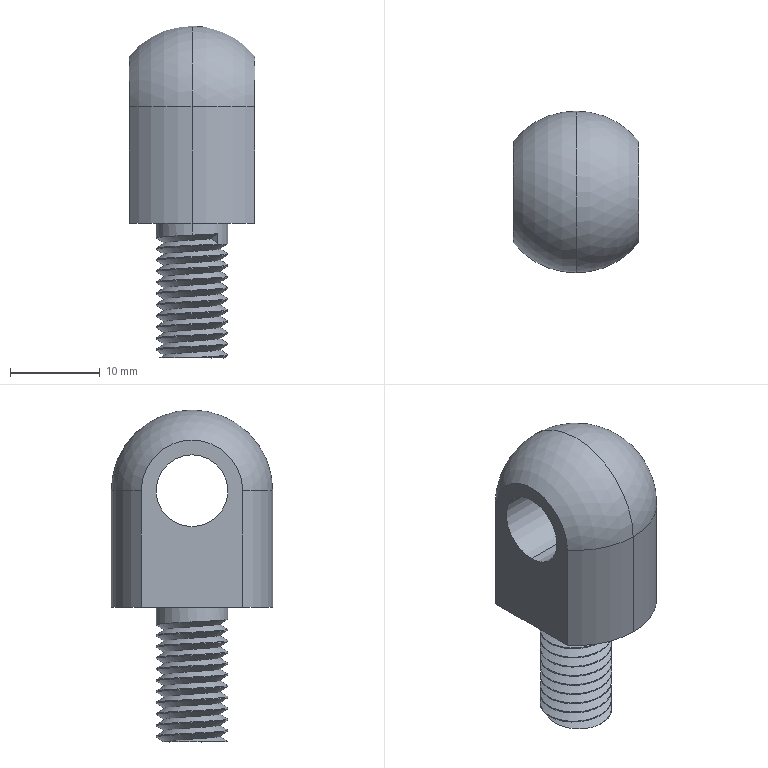Component | SolidWorks | HingeAssembly-3_Hinge2-1 | 1 solid | 38 faces | volume 4252 mm3 | cylinder 28 | plane 6 | sphere 2 | spline 2 | commonest cylinder face diameters 8 x25 18 x3